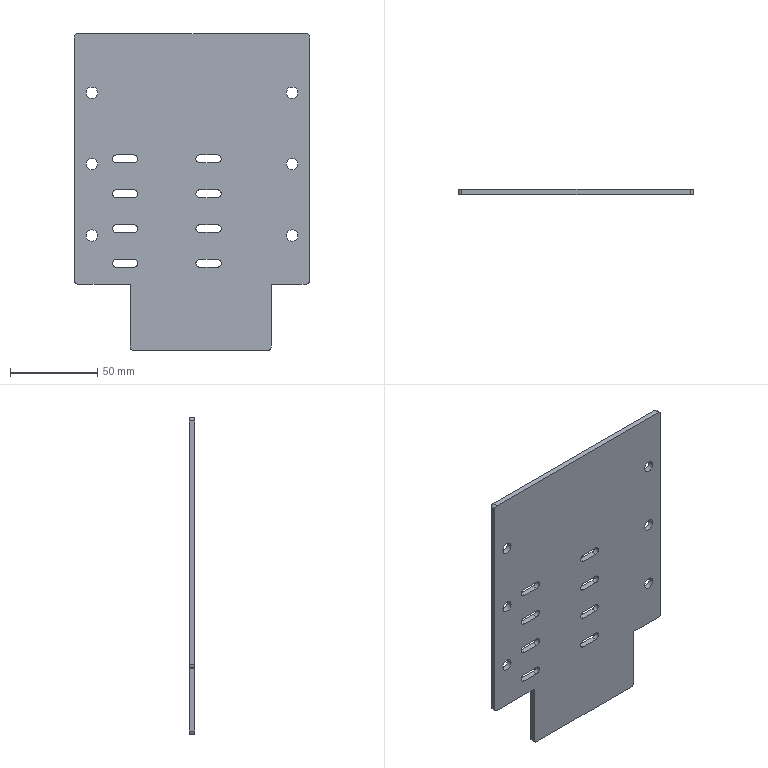Component | SolidWorks | B-TRD899MINI-2213-02DesiccantBasePlate-1 | 1 solid | 68 faces | volume 65461 mm3 | cylinder 42 | plane 26 | commonest cylinder face diameters 4.5 x24 6.6 x12 4 x6 | material SUS201